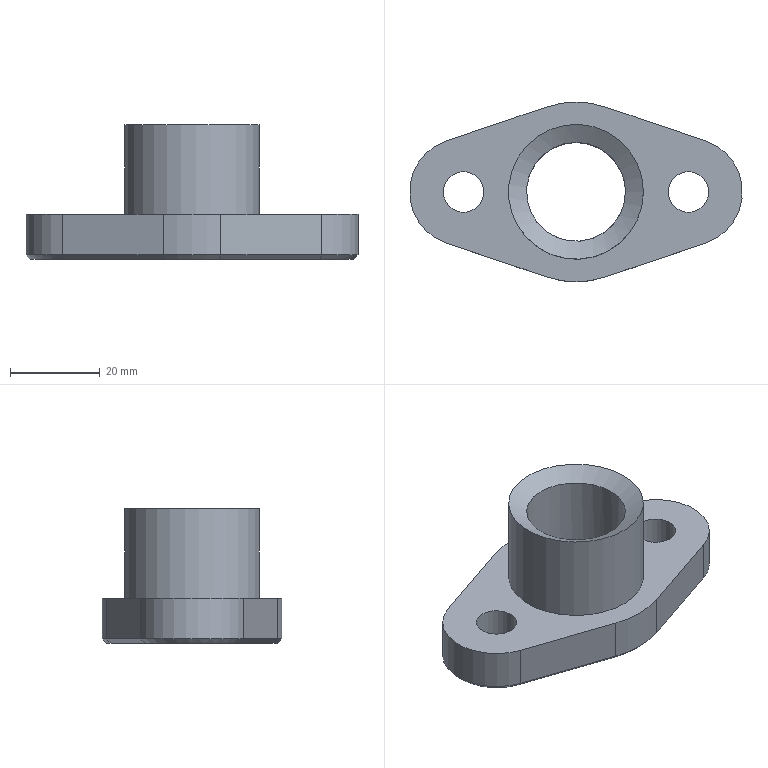Component | NX | 9_PACKING_GLAND | 1 solid | 24 faces | volume 22217 mm3 | plane 10 | cylinder 8 | cone 6 | commonest cylinder face diameters 24 x2 40 x2 9 x2 30 x1 22 x1